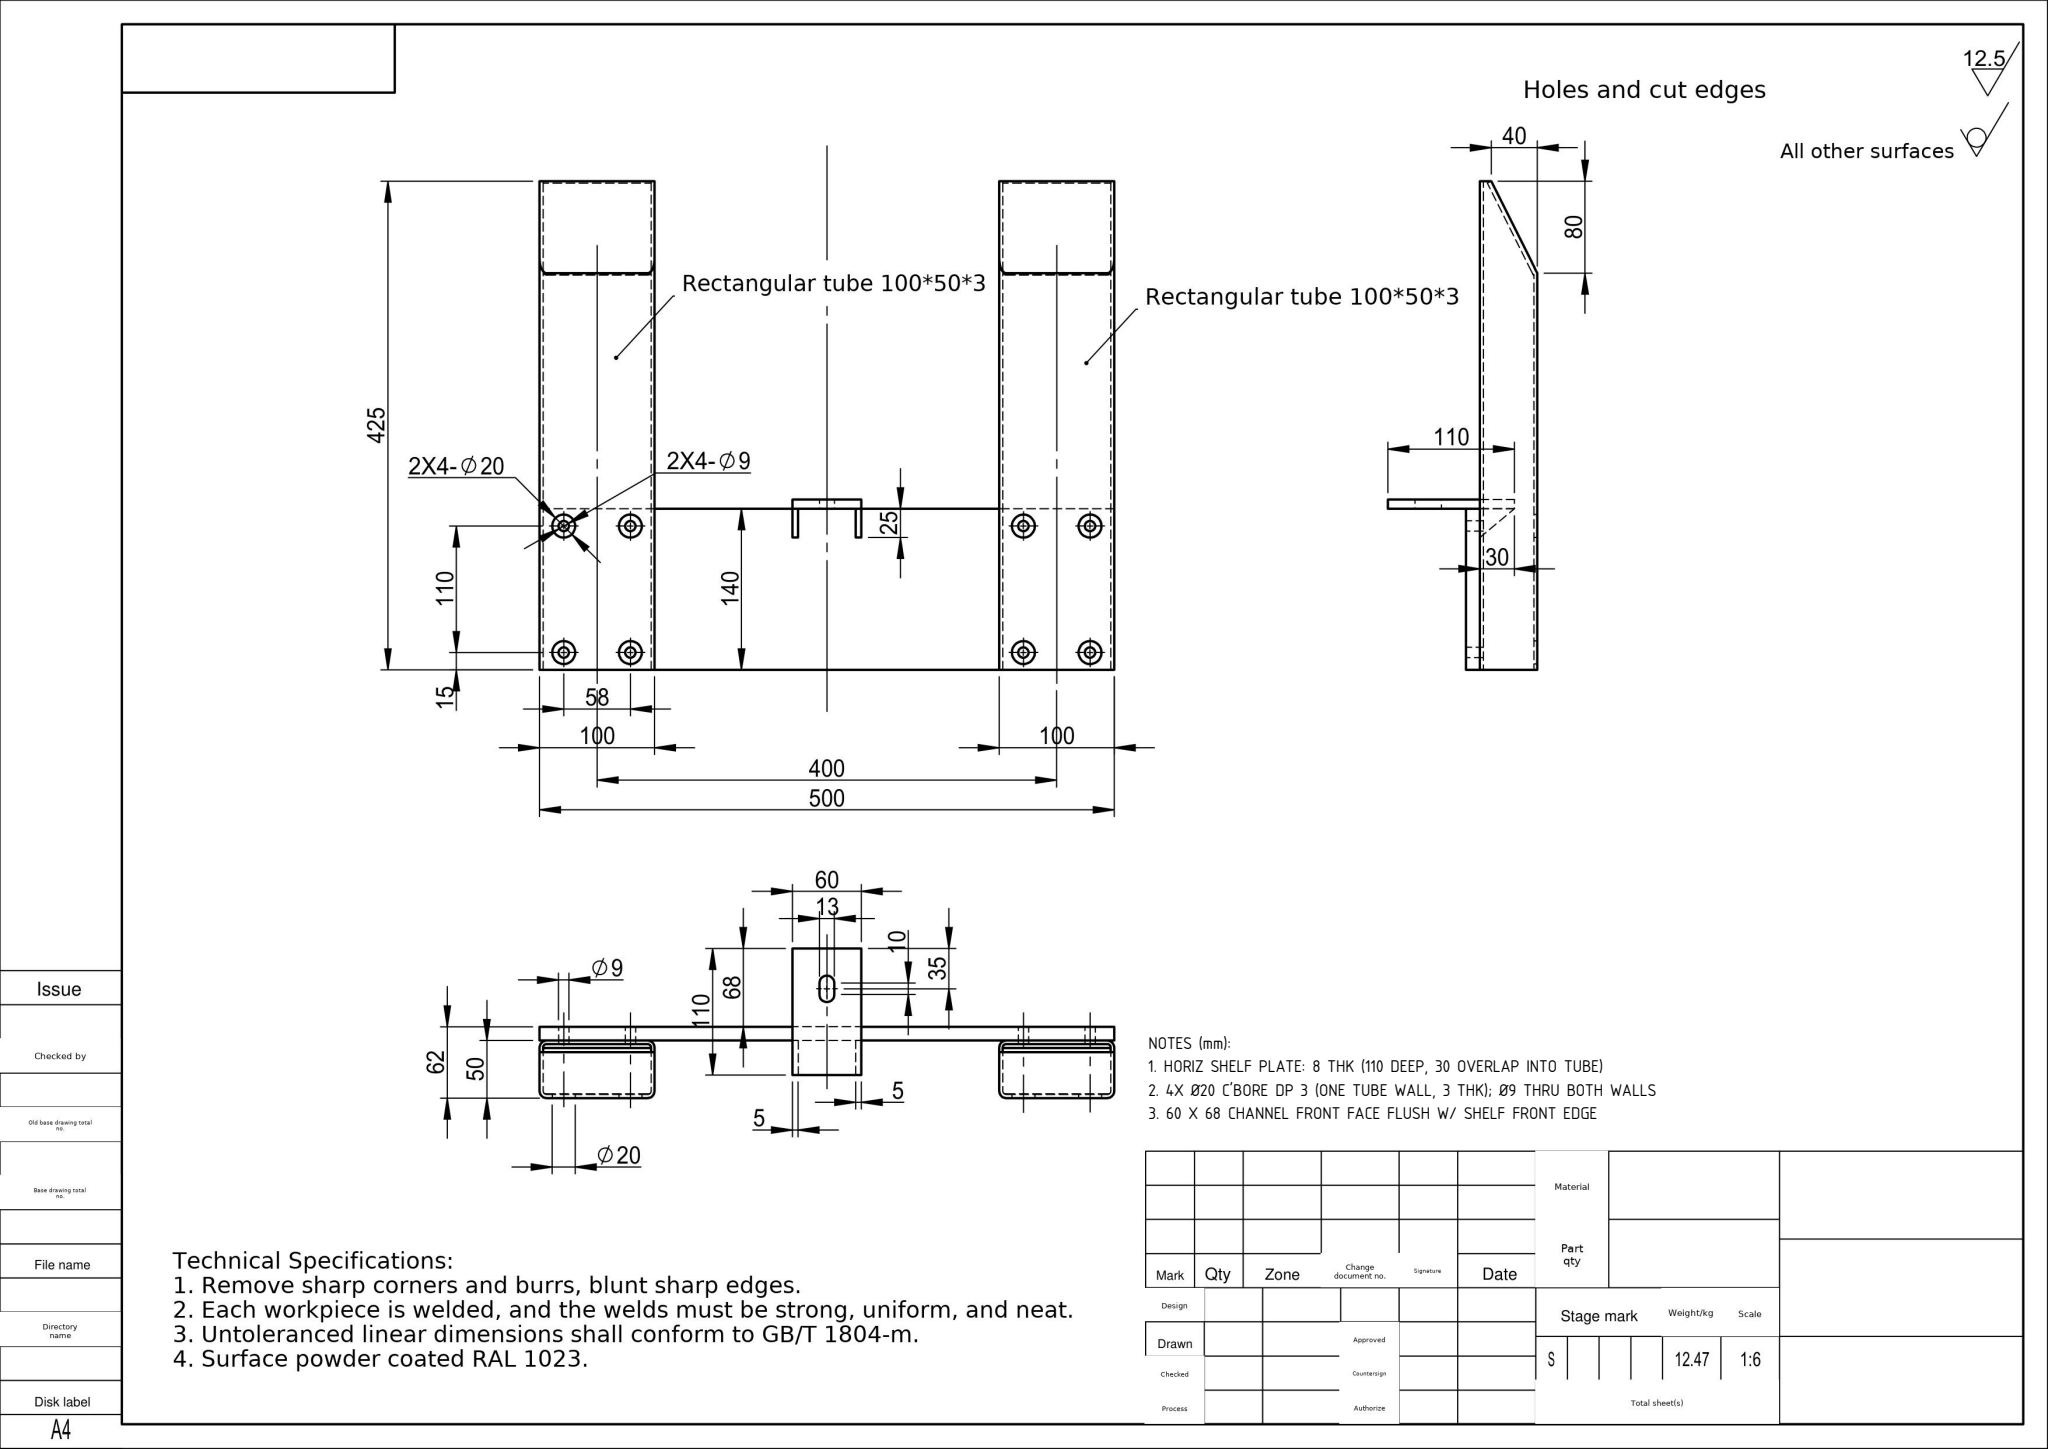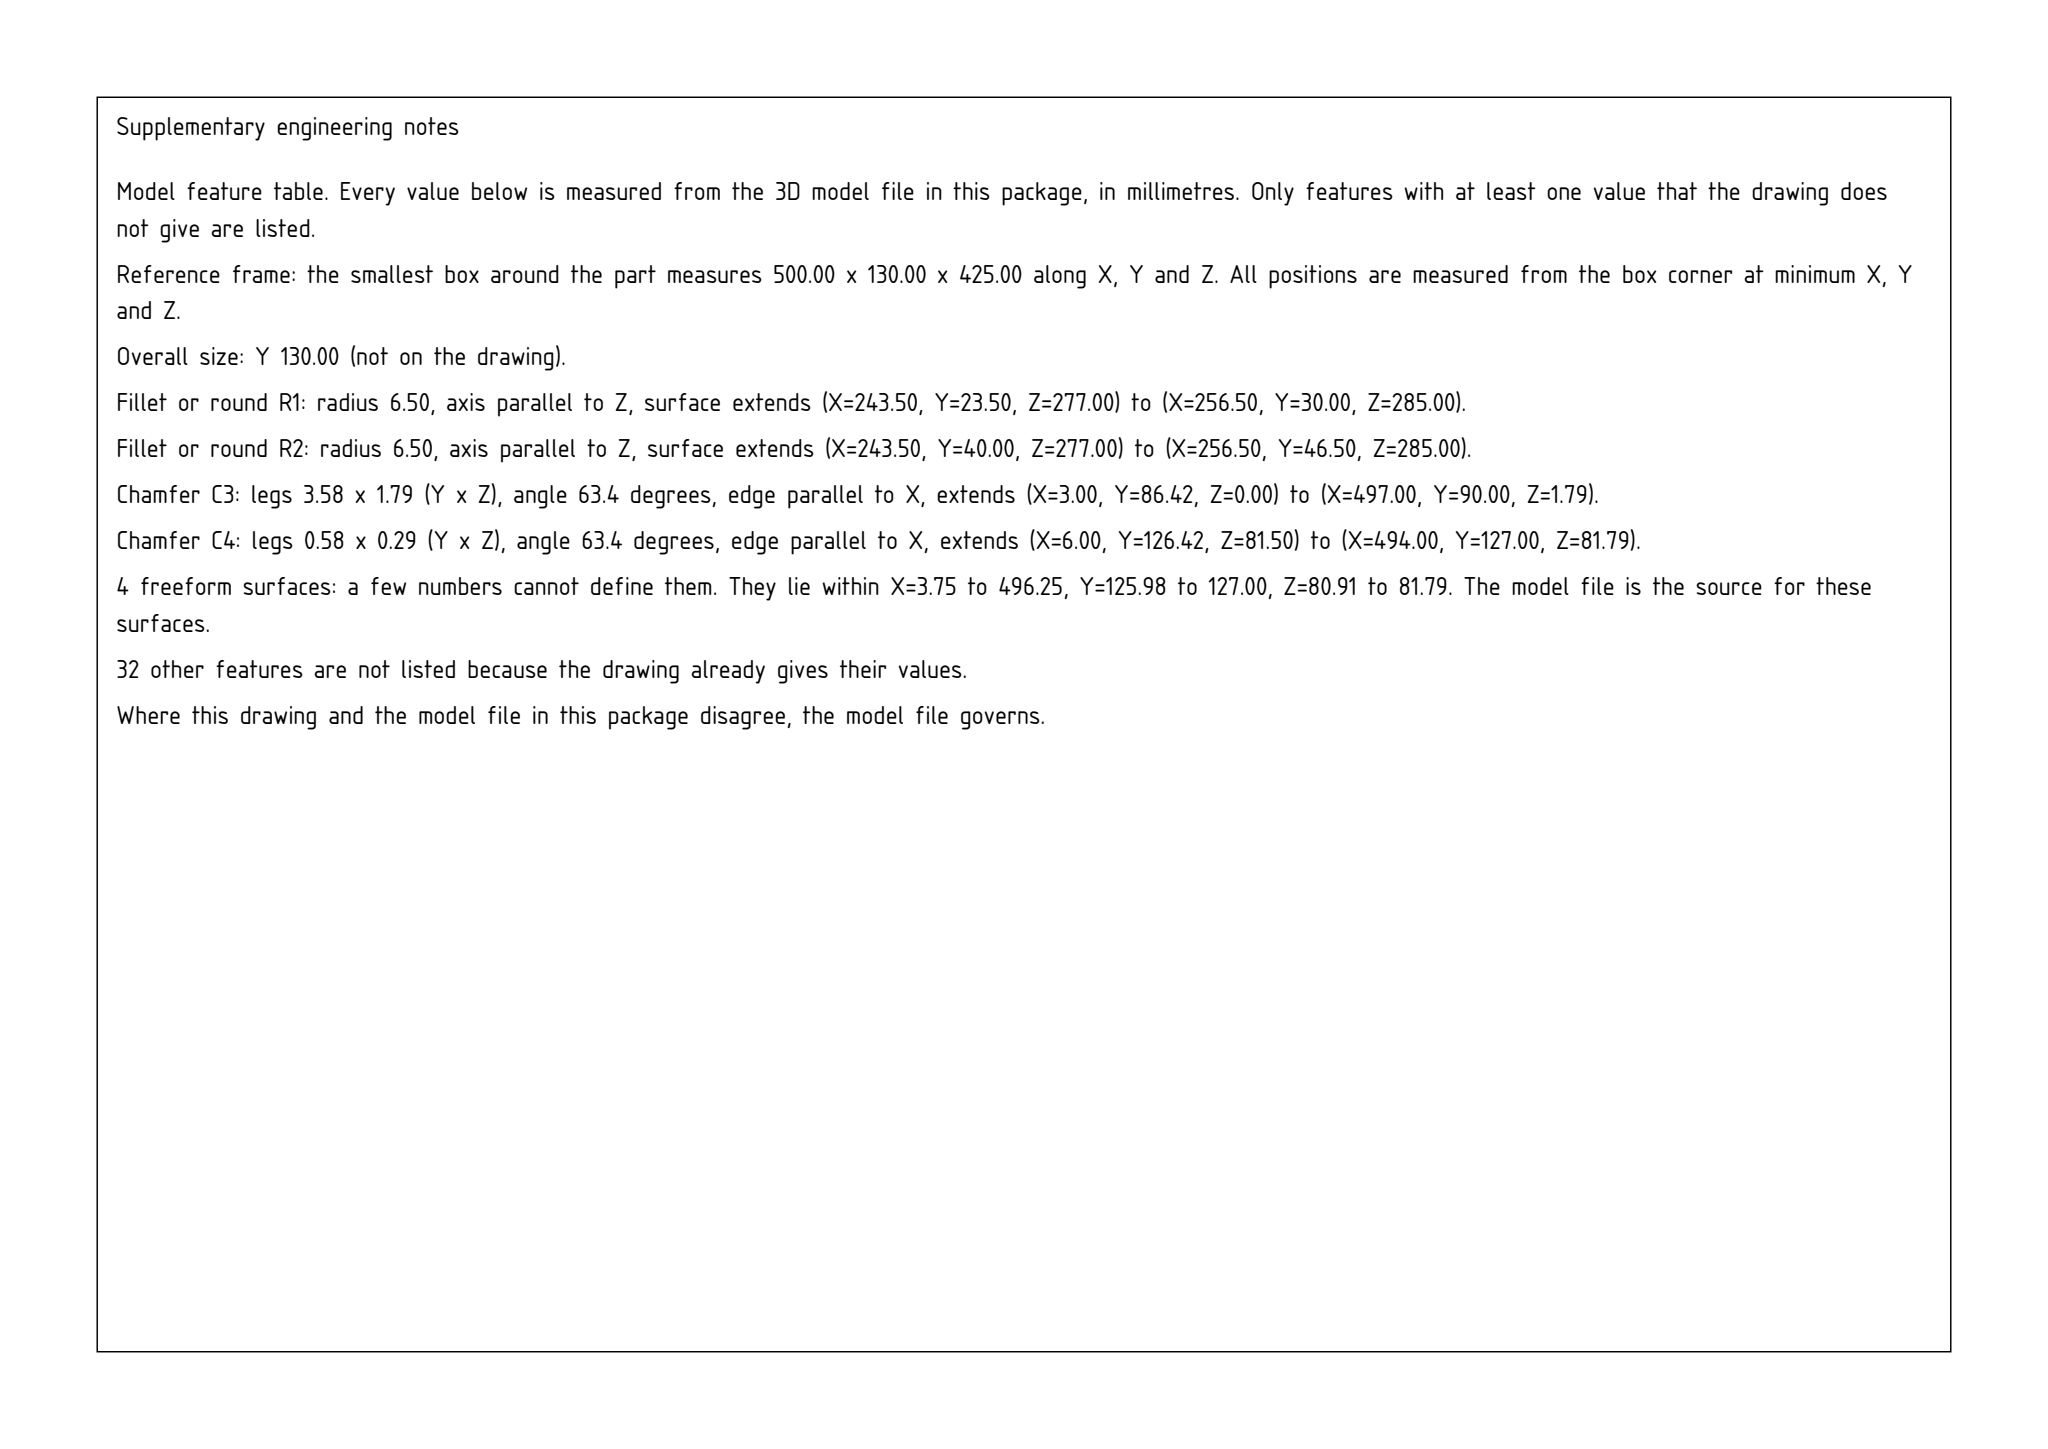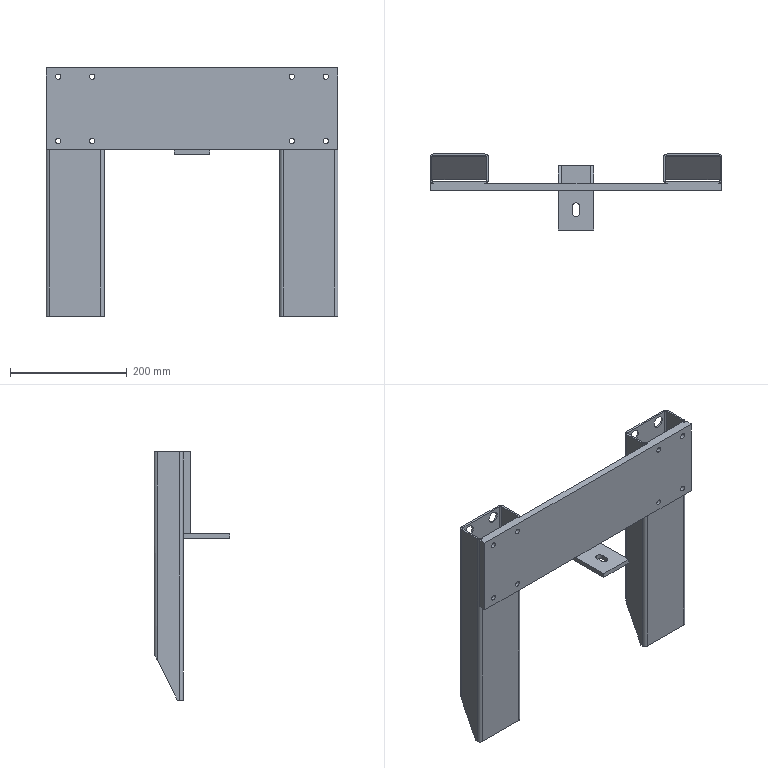Part | SolidWorks | mm | 1 solid | 102 faces | box 500 x 130 x 425 mm | volume 1598253 mm3 | cylinder 50 | plane 48 | spline 4 | commonest cylinder face diameters 9 x16 20 x16 12 x8 6 x8 13 x2
Drawing notes:
HORIZ SHELF PLATE: 8 THK (110 DEEP, 30 OVERLAP INTO TUBE) | from the solid: z-planes at 277.0 and 285.0 bound shelf plate => 8 mm thickness
4X Ø20 C'BORE DP 3 (ONE TUBE WALL, 3 THK); Ø9 THRU BOTH WALLS | from the solid: Ø20 y-axis cyls length 3.0 at (21/79/421/479, z300/410); Ø9 y-axis cyls length 15.0 same locations
60 X 68 CHANNEL FRONT FACE FLUSH W/ SHELF FRONT EDGE | from the solid: channel x-planes 220/225/275/280; y-planes 0 and 68 vs shelf front edge y=0
build123d program:
from build123d import *

# Parameters (mm, degrees)
SKETCH1_2_W                                   = 500
SKETCH1_2_H                                   = 140
BOSS_EXTRUDE1_DEPTH                           = 12
GB_6728_1986_RECTANGULAR_HOLLOW_SECTION_DEPTH = 425
GB_6728_1986_RECTANGULAR_HOLLOW_SECT_2_DEPTH  = 425
SKETCH9_R                                     = 10
CUT_EXTRUDE2_DEPTH                            = 10
SKETCH10_R                                    = 4.5
CUT_EXTRUDE3_DEPTH                            = 439.599
SKETCH11_W                                    = 60
SKETCH11_H                                    = 110
BOSS_EXTRUDE5_DEPTH                           = 8
GUSSET1_THICKNESS                             = 5
GUSSET2_THICKNESS                             = 5
CUT_EXTRUDE4_DEPTH                            = 617.968
BOSS_EXTRUDE6_DEPTH                           = 4


with BuildPart() as part:
    # Sketch1_2 → Boss-Extrude1 (new body)
    with BuildSketch(Plane(origin=(0, 0, 0), x_dir=(1, 0, 0), z_dir=(0, 1, 0))):
        Rectangle(SKETCH1_2_W, SKETCH1_2_H)
    extrude(amount=BOSS_EXTRUDE1_DEPTH)


with BuildPart() as body_2:
    # Sketch1 → GB_6728-1986 Rectangular Hollow Section (new body)
    with BuildSketch(Plane(origin=(-200, 37, 70), x_dir=(0, 1, 0), z_dir=(0, 0, -1))):
        with BuildLine():
            Line((-19, -50), (19, -50))
            ThreePointArc((19, -50), (23.243, -48.243), (25, -44))
            Line((25, -44), (25, 44))
            ThreePointArc((25, 44), (23.243, 48.243), (19, 50))
            Line((19, 50), (-19, 50))
            ThreePointArc((-19, 50), (-23.243, 48.243), (-25, 44))
            Line((-25, 44), (-25, -44))
            ThreePointArc((-25, -44), (-23.243, -48.243), (-19, -50))
        make_face()
        with BuildLine():
            Line((-19, -47), (19, -47))
            ThreePointArc((19, -47), (21.121, -46.121), (22, -44))
            Line((22, -44), (22, 44))
            ThreePointArc((22, 44), (21.121, 46.121), (19, 47))
            Line((19, 47), (-19, 47))
            ThreePointArc((-19, 47), (-21.121, 46.121), (-22, 44))
            Line((-22, 44), (-22, -44))
            ThreePointArc((-22, -44), (-21.121, -46.121), (-19, -47))
        make_face(mode=Mode.SUBTRACT)
    extrude(amount=GB_6728_1986_RECTANGULAR_HOLLOW_SECTION_DEPTH)


with BuildPart() as body_3:
    # Sketch1 on segment 2 (on carried to segment 2) → GB_6728-1986 Rectangular Hollow Sect 2 (new body)
    with BuildSketch(Plane(origin=(200, 37, 70), x_dir=(0, 1, 0), z_dir=(0, 0, -1))):
        with BuildLine():
            Line((-19, -50), (19, -50))
            ThreePointArc((19, -50), (23.243, -48.243), (25, -44))
            Line((25, -44), (25, 44))
            ThreePointArc((25, 44), (23.243, 48.243), (19, 50))
            Line((19, 50), (-19, 50))
            ThreePointArc((-19, 50), (-23.243, 48.243), (-25, 44))
            Line((-25, 44), (-25, -44))
            ThreePointArc((-25, -44), (-23.243, -48.243), (-19, -50))
        make_face()
        with BuildLine():
            Line((-19, -47), (19, -47))
            ThreePointArc((19, -47), (21.121, -46.121), (22, -44))
            Line((22, -44), (22, 44))
            ThreePointArc((22, 44), (21.121, 46.121), (19, 47))
            Line((19, 47), (-19, 47))
            ThreePointArc((-19, 47), (-21.121, 46.121), (-22, 44))
            Line((-22, 44), (-22, -44))
            ThreePointArc((-22, -44), (-21.121, -46.121), (-19, -47))
        make_face(mode=Mode.SUBTRACT)
    extrude(amount=GB_6728_1986_RECTANGULAR_HOLLOW_SECT_2_DEPTH)


with BuildPart() as cut_extrude2_tool:
    # Sketch9 → Cut-Extrude2 (new body)
    with BuildSketch(Plane(origin=(0, 62, 0), x_dir=(1, 0, 0), z_dir=(0, 1, 0))):
        with Locations(Location((171, -55, 0), (0, 0, 180))):
            Circle(SKETCH9_R)
        with Locations(Location((229, -55, 0), (0, 0, 180))):
            Circle(SKETCH9_R)
        with Locations(Location((171, 55, 0), (0, 0, 180))):
            Circle(SKETCH9_R)
        with Locations(Location((229, 55, 0), (0, 0, 180))):
            Circle(SKETCH9_R)
        with Locations((-229, 55)):
            Circle(SKETCH9_R)
        with Locations((-171, 55)):
            Circle(SKETCH9_R)
        with Locations((-229, -55)):
            Circle(SKETCH9_R)
        with Locations((-171, -55)):
            Circle(SKETCH9_R)
    extrude(amount=-CUT_EXTRUDE2_DEPTH)


with BuildPart() as body_2_1:
    add(body_2.part)

    # Cut-Extrude2: cut by cut_extrude2_tool
    add(cut_extrude2_tool.part, mode=Mode.SUBTRACT)


with BuildPart() as body_3_1:
    add(body_3.part)

    # Cut-Extrude2: cut by cut_extrude2_tool
    add(cut_extrude2_tool.part, mode=Mode.SUBTRACT)


with BuildPart() as cut_extrude3_tool:
    # Sketch10 → Cut-Extrude3 (new, through all)
    with BuildSketch(Plane(origin=(0, 62, 0), x_dir=(1, 0, 0), z_dir=(0, 1, 0))):
        with Locations(Location((-229, 55, 0), (0, 0, 180))):
            Circle(SKETCH10_R)
        with Locations(Location((-171, 55, 0), (0, 0, 180))):
            Circle(SKETCH10_R)
        with Locations(Location((-229, -55, 0), (0, 0, 180))):
            Circle(SKETCH10_R)
        with Locations(Location((-171, -55, 0), (0, 0, 180))):
            Circle(SKETCH10_R)
        with Locations(Location((171, 55, 0), (0, 0, 180))):
            Circle(SKETCH10_R)
        with Locations(Location((229, 55, 0), (0, 0, 180))):
            Circle(SKETCH10_R)
        with Locations(Location((171, -55, 0), (0, 0, 180))):
            Circle(SKETCH10_R)
        with Locations(Location((229, -55, 0), (0, 0, 180))):
            Circle(SKETCH10_R)
    extrude(amount=-CUT_EXTRUDE3_DEPTH)


with BuildPart() as part_1:
    add(part.part)

    # Cut-Extrude3: cut by cut_extrude3_tool
    add(cut_extrude3_tool.part, mode=Mode.SUBTRACT)


with BuildPart() as body_2_2:
    add(body_2_1.part)

    # Cut-Extrude3: cut by cut_extrude3_tool
    add(cut_extrude3_tool.part, mode=Mode.SUBTRACT)


with BuildPart() as body_3_2:
    add(body_3_1.part)

    # Cut-Extrude3: cut by cut_extrude3_tool
    add(cut_extrude3_tool.part, mode=Mode.SUBTRACT)


with BuildPart() as body_4:
    # Sketch11 → Boss-Extrude5 (new body)
    with BuildSketch(Plane(origin=(0, 0, -70), x_dir=(-1, 0, 0), z_dir=(0, 0, -1))):
        with Locations((0, -13)):
            Rectangle(SKETCH11_W, SKETCH11_H)
        with BuildLine():
            Line((-6.5, -38), (-6.5, -28))
            ThreePointArc((-6.5, -28), (0, -21.5), (6.5, -28))
            Line((6.5, -28), (6.5, -38))
            ThreePointArc((6.5, -38), (0, -44.5), (-6.5, -38))
        make_face(mode=Mode.SUBTRACT)
    extrude(amount=BOSS_EXTRUDE5_DEPTH)


with BuildPart() as body_5:
    # Gusset1: a gusset: a plate 5.0 thick in the corner of two members, its outline drawn in place
    gusset1_outline = Wire([Line((30, 12, -70), (30, 42, -70)), Line((30, 42, -70), (30, 12, -45)), Line((30, 12, -45), (30, 12, -70))])
    add(extrude(Face(gusset1_outline), amount=GUSSET1_THICKNESS, dir=(-1, 0, 0)))


with BuildPart() as body_6:
    # Gusset2: a gusset: a plate 5.0 thick in the corner of two members, its outline drawn in place
    gusset2_outline = Wire([Line((-25, 12, -70), (-25, 42, -70)), Line((-25, 42, -70), (-25, 12, -45)), Line((-25, 12, -45), (-25, 12, -70))])
    add(extrude(Face(gusset2_outline), amount=GUSSET2_THICKNESS, dir=(-1, 0, 0)))


with BuildPart() as cut_extrude4_tool:
    # Sketch14 → Cut-Extrude4 (new, through all)
    with BuildSketch(Plane.ZY.offset(250)):
        Polygon((-355, 62), (-275, 62), (-355, 22), align=None)
    extrude(amount=-CUT_EXTRUDE4_DEPTH)


with BuildPart() as body_2_3:
    add(body_2_2.part)

    # Cut-Extrude4: cut by cut_extrude4_tool
    add(cut_extrude4_tool.part, mode=Mode.SUBTRACT)



with BuildPart() as body_3_3:
    add(body_3_2.part)

    # Cut-Extrude4: cut by cut_extrude4_tool
    add(cut_extrude4_tool.part, mode=Mode.SUBTRACT)


with BuildPart() as body_2_4:
    add(body_2_3.part)

    add(body_3_3.part)  # Boss-Extrude6 merges body 3
    # Sketch15 → Boss-Extrude6 (add)
    with BuildSketch(Plane(origin=(0, 159.6, -79.8), x_dir=(1, 0, 0), z_dir=(0, 0.8944, -0.4472))):
        with BuildLine():
            Line((150, 307.683), (250, 307.683))
            Line((250, 307.683), (250, 231.657))
            add(Edge.make_bspline(
                [(244, 218.24), (250, 218.24), (250, 231.657)],
                knots=[0, 0, 0, 1.571, 1.571, 1.571], degree=2, weights=[1, 0.7071, 1]))
            Line((244, 218.24), (156, 218.24))
            add(Edge.make_bspline(
                [(150, 231.657), (150, 218.24), (156, 218.24)],
                knots=[4.712, 4.712, 4.712, 6.283, 6.283, 6.283], degree=2, weights=[1, 0.7071, 1]))
            Line((150, 231.657), (150, 307.683))
        make_face()
        with BuildLine():
            Line((-250, 307.683), (-150, 307.683))
            Line((-150, 307.683), (-150, 231.657))
            add(Edge.make_bspline(
                [(-156, 218.24), (-150, 218.24), (-150, 231.657)],
                knots=[0, 0, 0, 1.571, 1.571, 1.571], degree=2, weights=[1, 0.7071, 1]))
            Line((-156, 218.24), (-244, 218.24))
            add(Edge.make_bspline(
                [(-250, 231.657), (-250, 218.24), (-244, 218.24)],
                knots=[4.712, 4.712, 4.712, 6.283, 6.283, 6.283], degree=2, weights=[1, 0.7071, 1]))
            Line((-250, 231.657), (-250, 307.683))
        make_face()
    extrude(amount=-BOSS_EXTRUDE6_DEPTH)


with BuildPart() as body_4_1:
    add(body_4.part)

    # Combine-RayDong-Repair: union body 2, body 6, part, body 5
    add(body_2_4.part)
    add(body_6.part)
    add(part_1.part)
    add(body_5.part)


solid = body_4_1.part